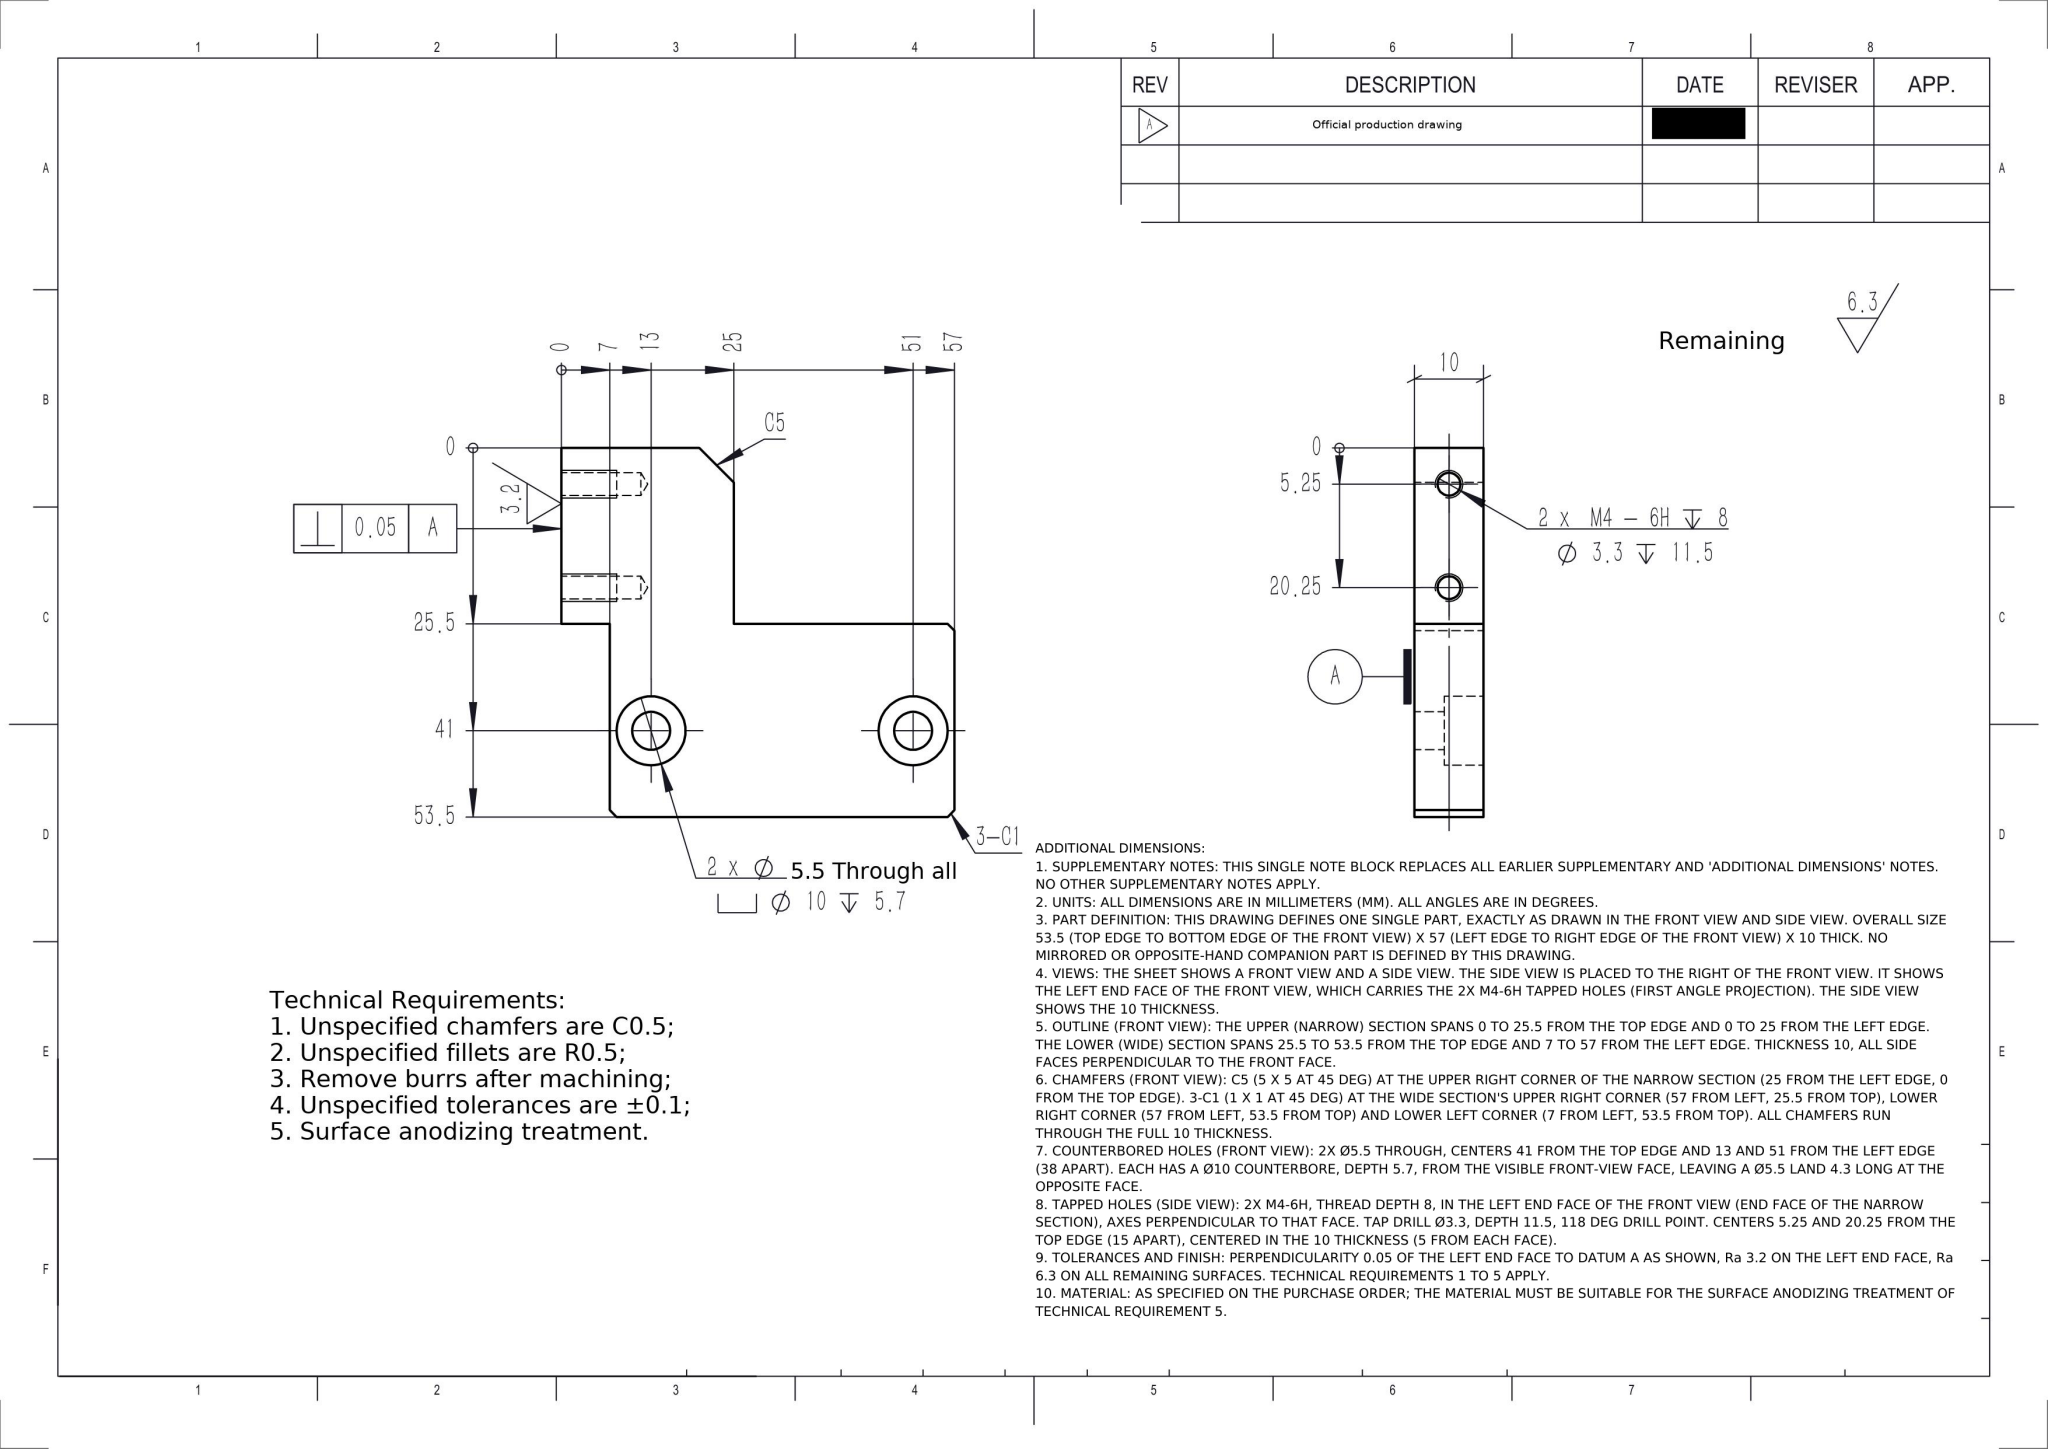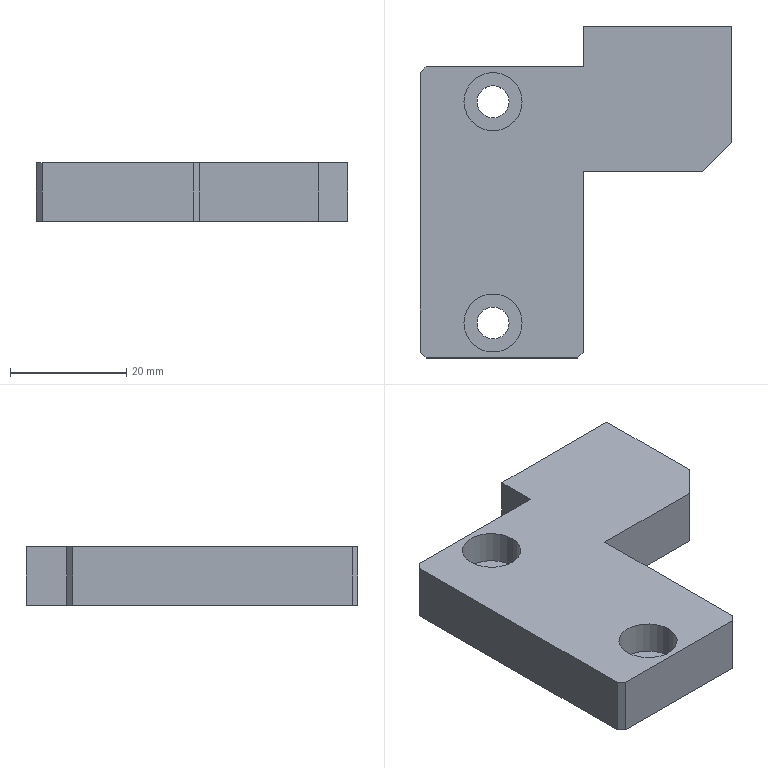Part | NX | mm | 1 solid | 32 faces | box 53.5 x 57 x 10 mm | volume 18933 mm3 | plane 16 | cylinder 12 | cone 4 | commonest cylinder face diameters 3.3 x4 10 x4 5.5 x4